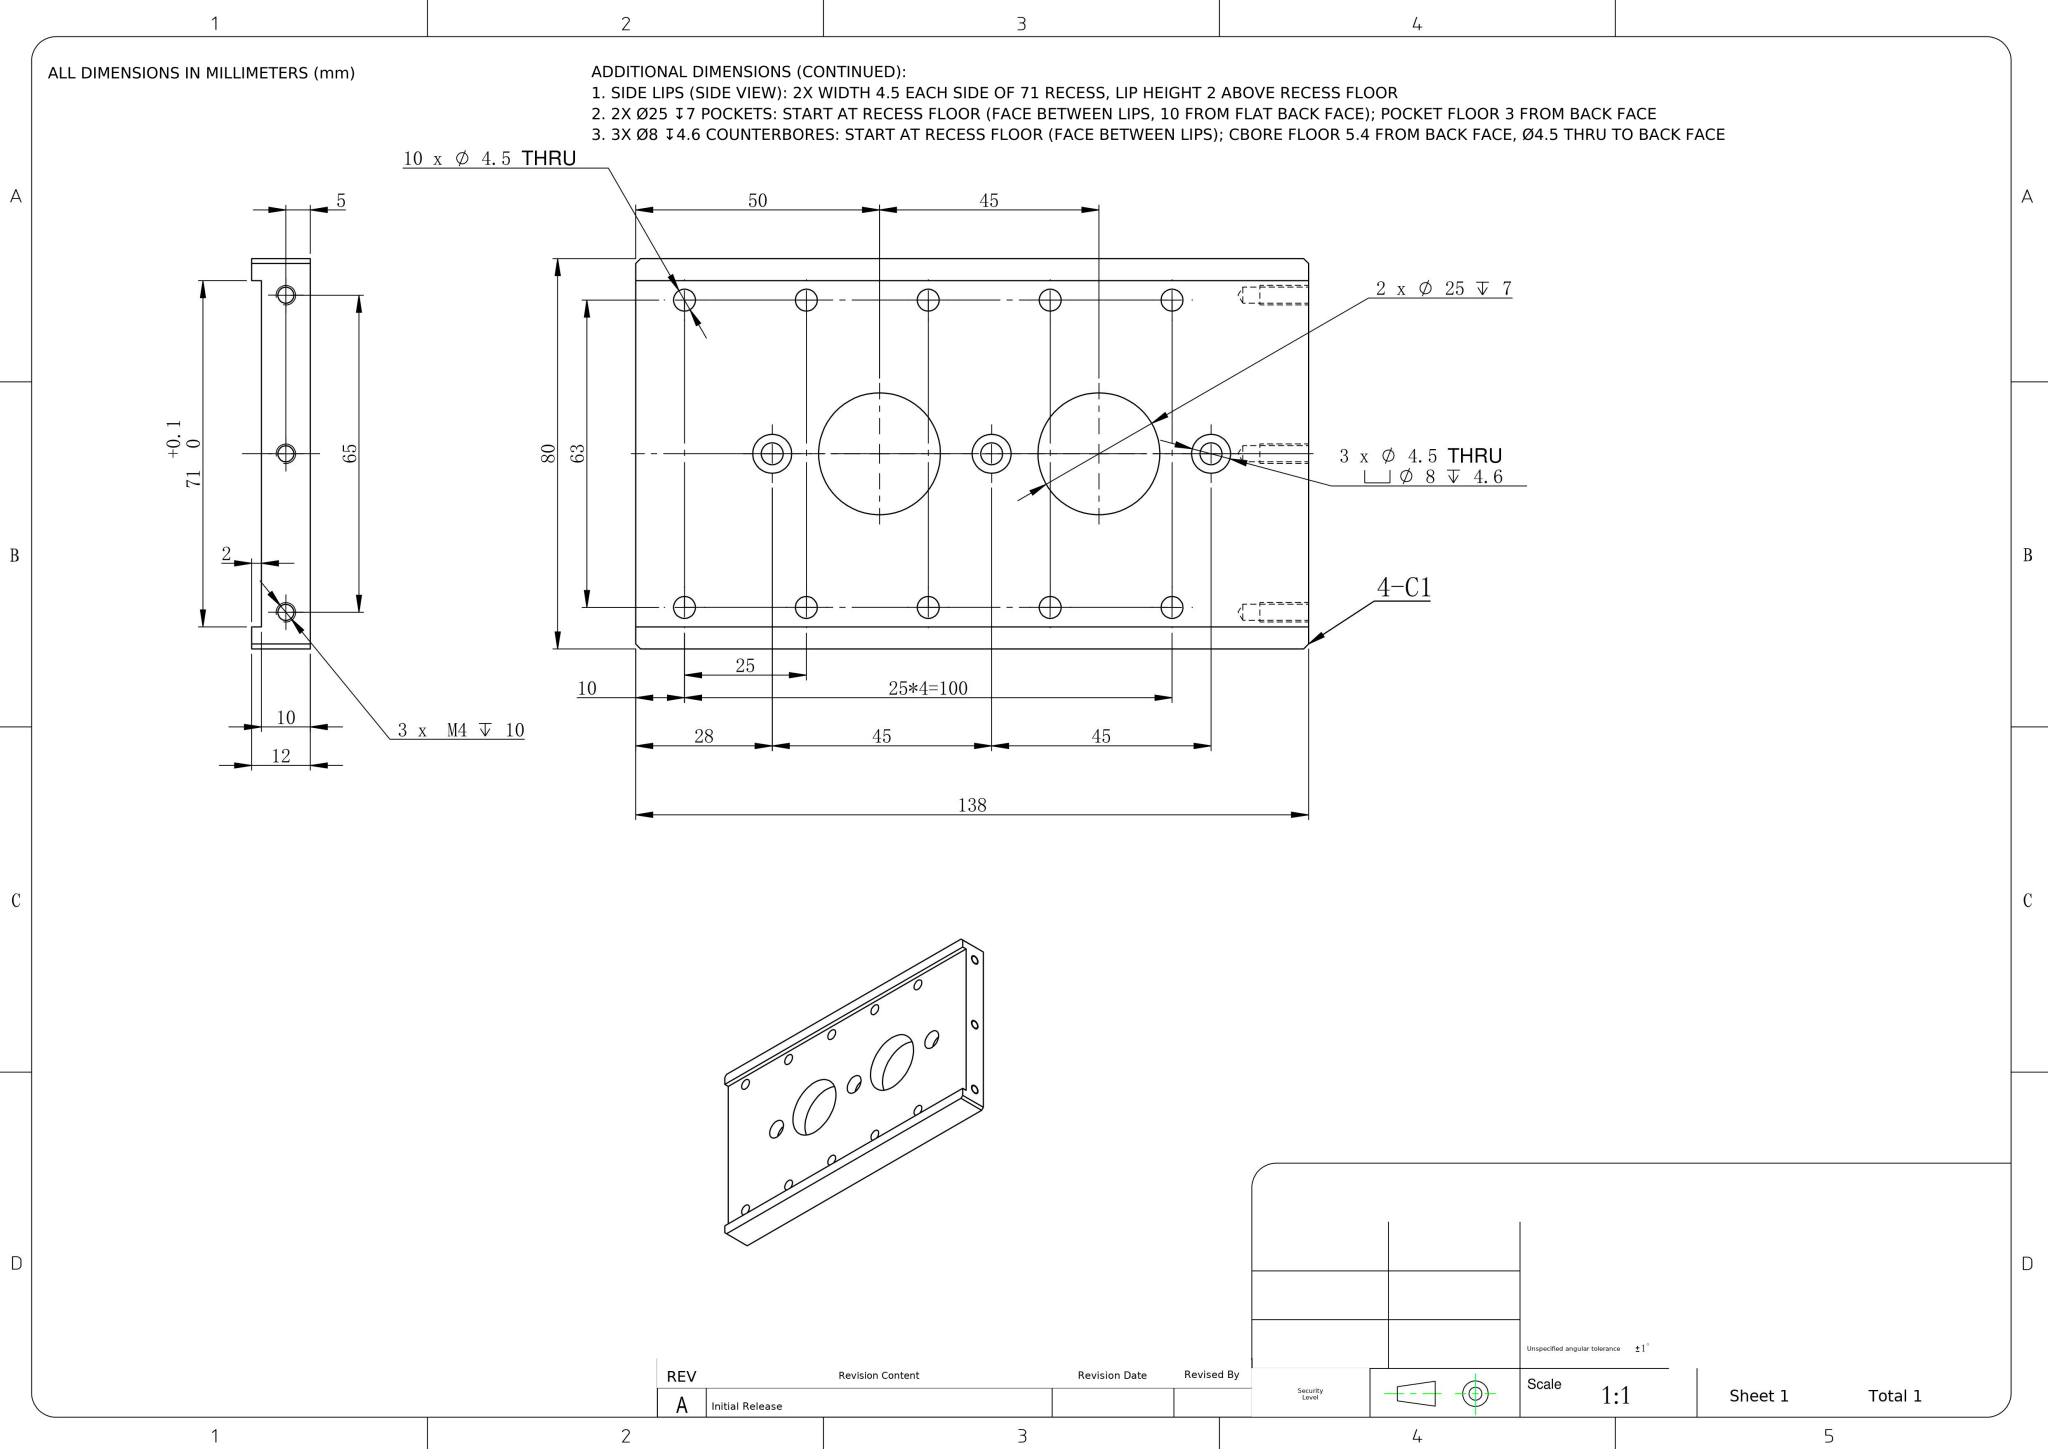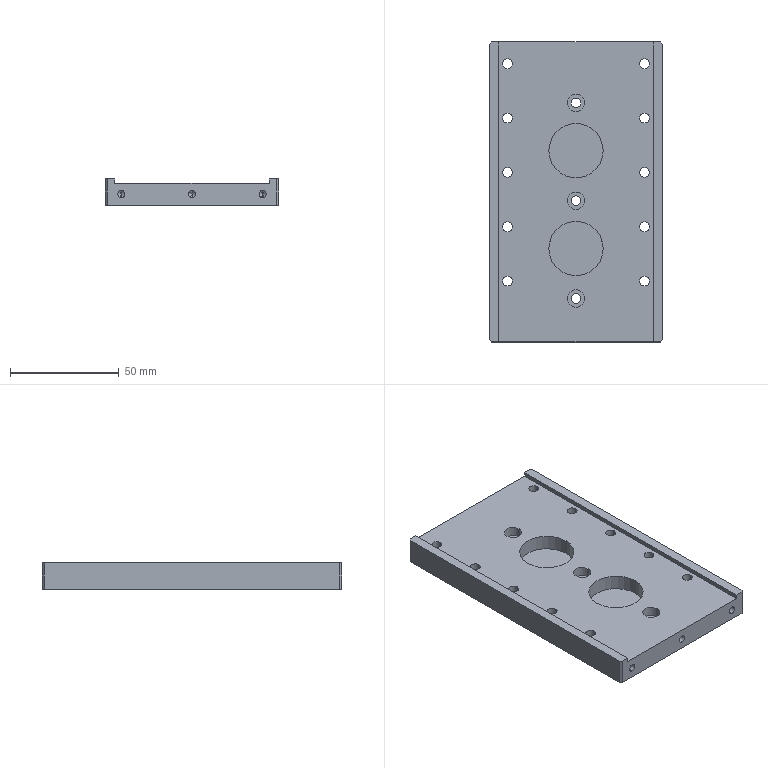Part | NX | mm | 1 solid | 67 faces | box 80 x 138 x 12 mm | volume 103091 mm3 | cylinder 42 | plane 19 | cone 6 | commonest cylinder face diameters 4.5 x26 8 x6 3.3 x6 25 x4